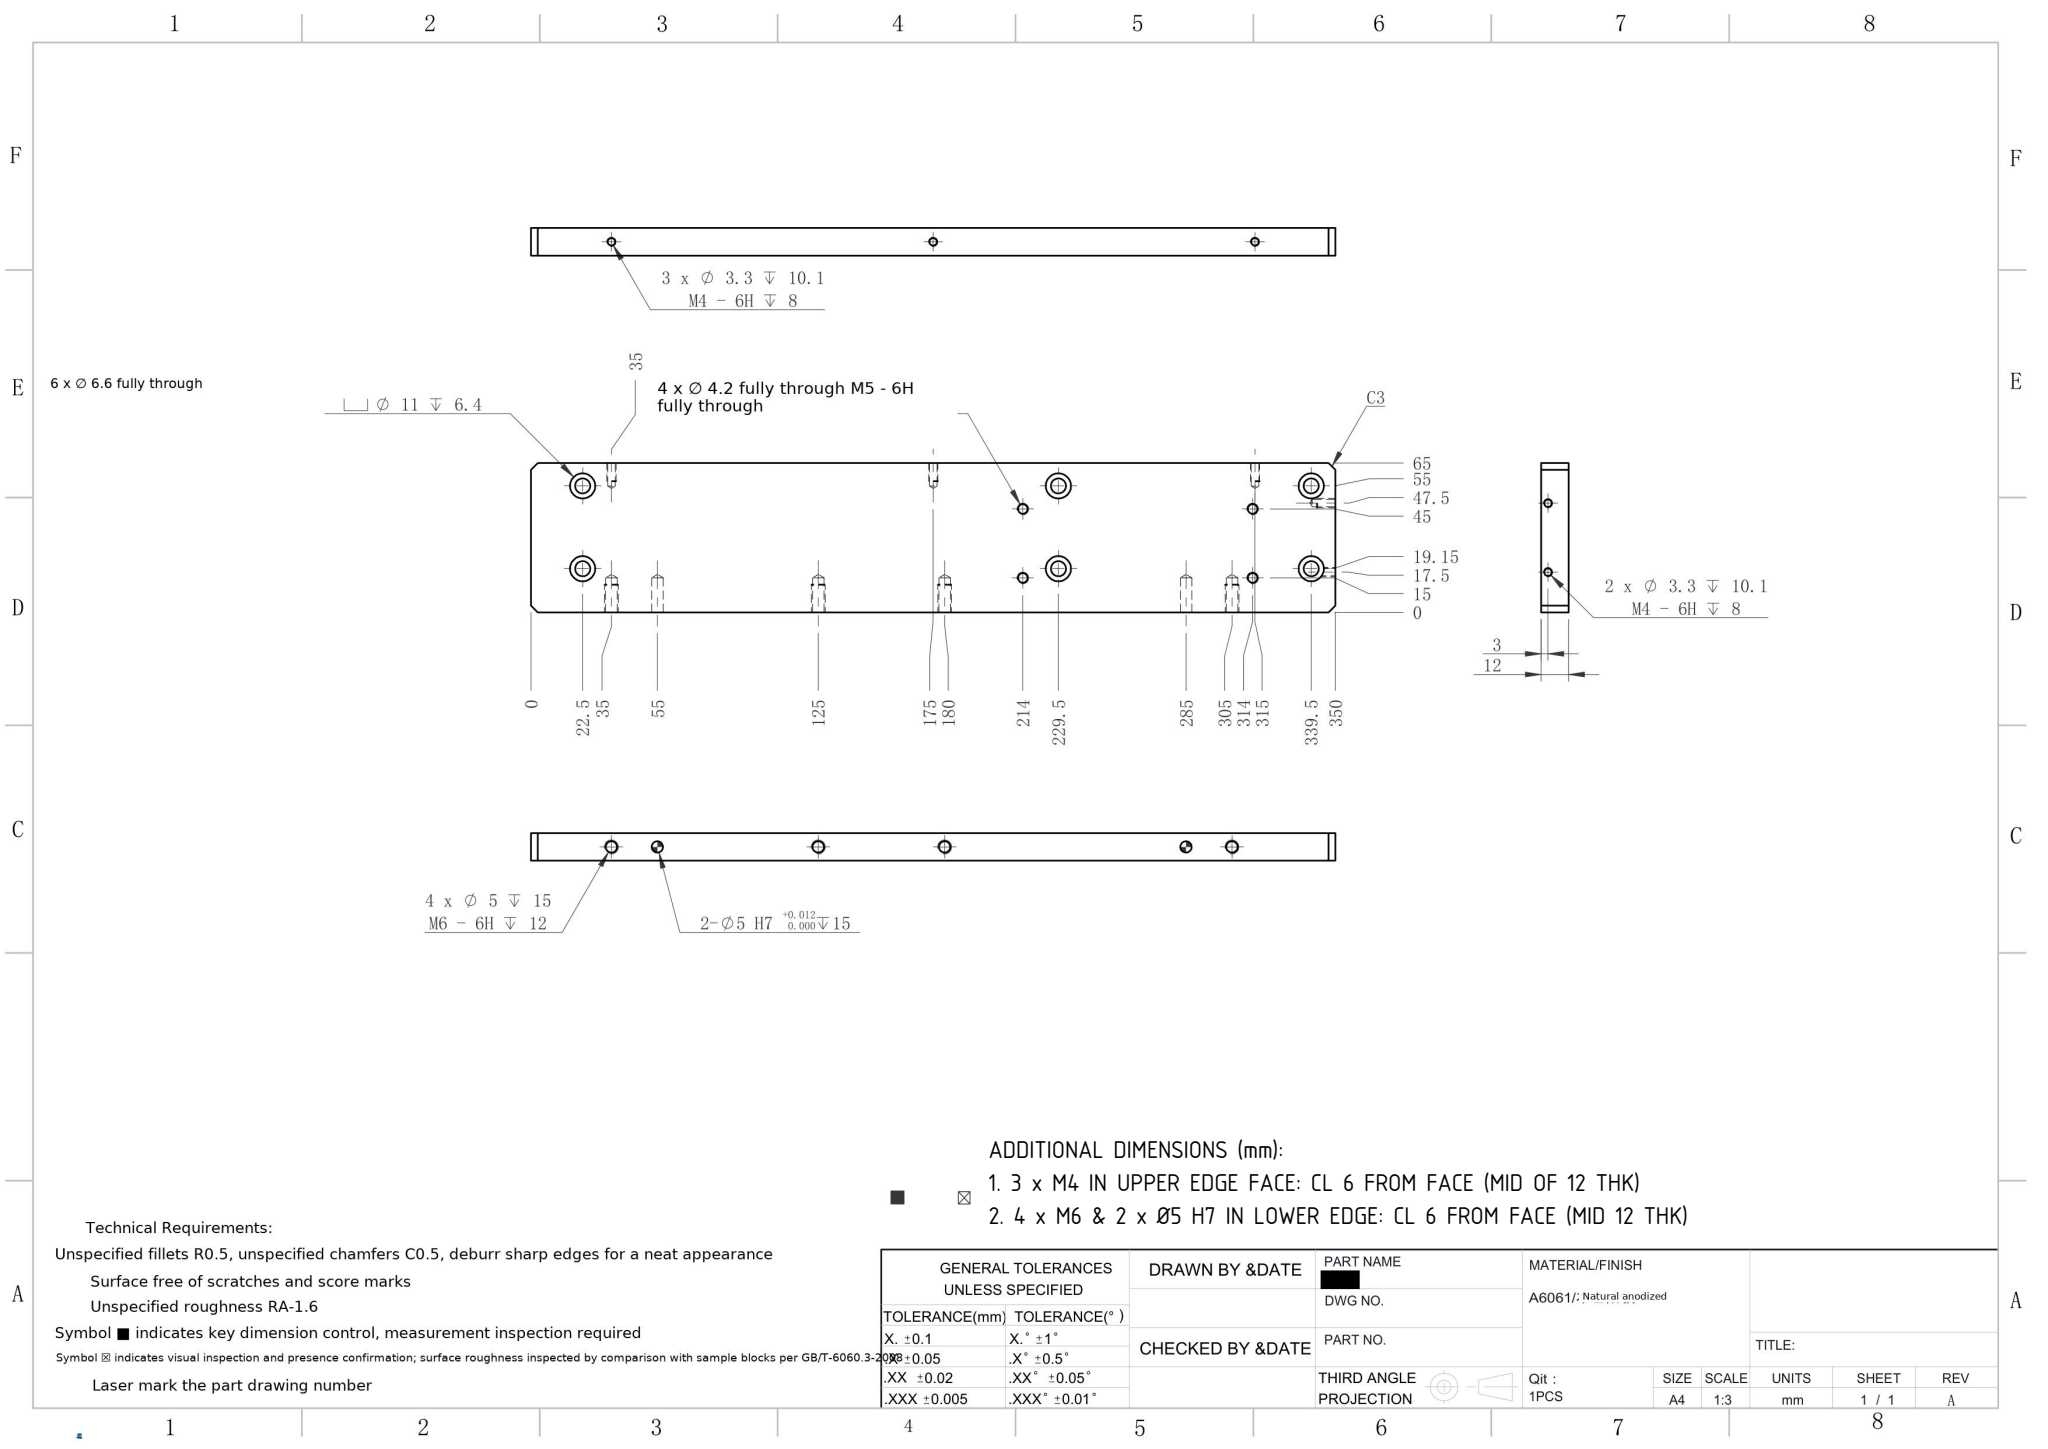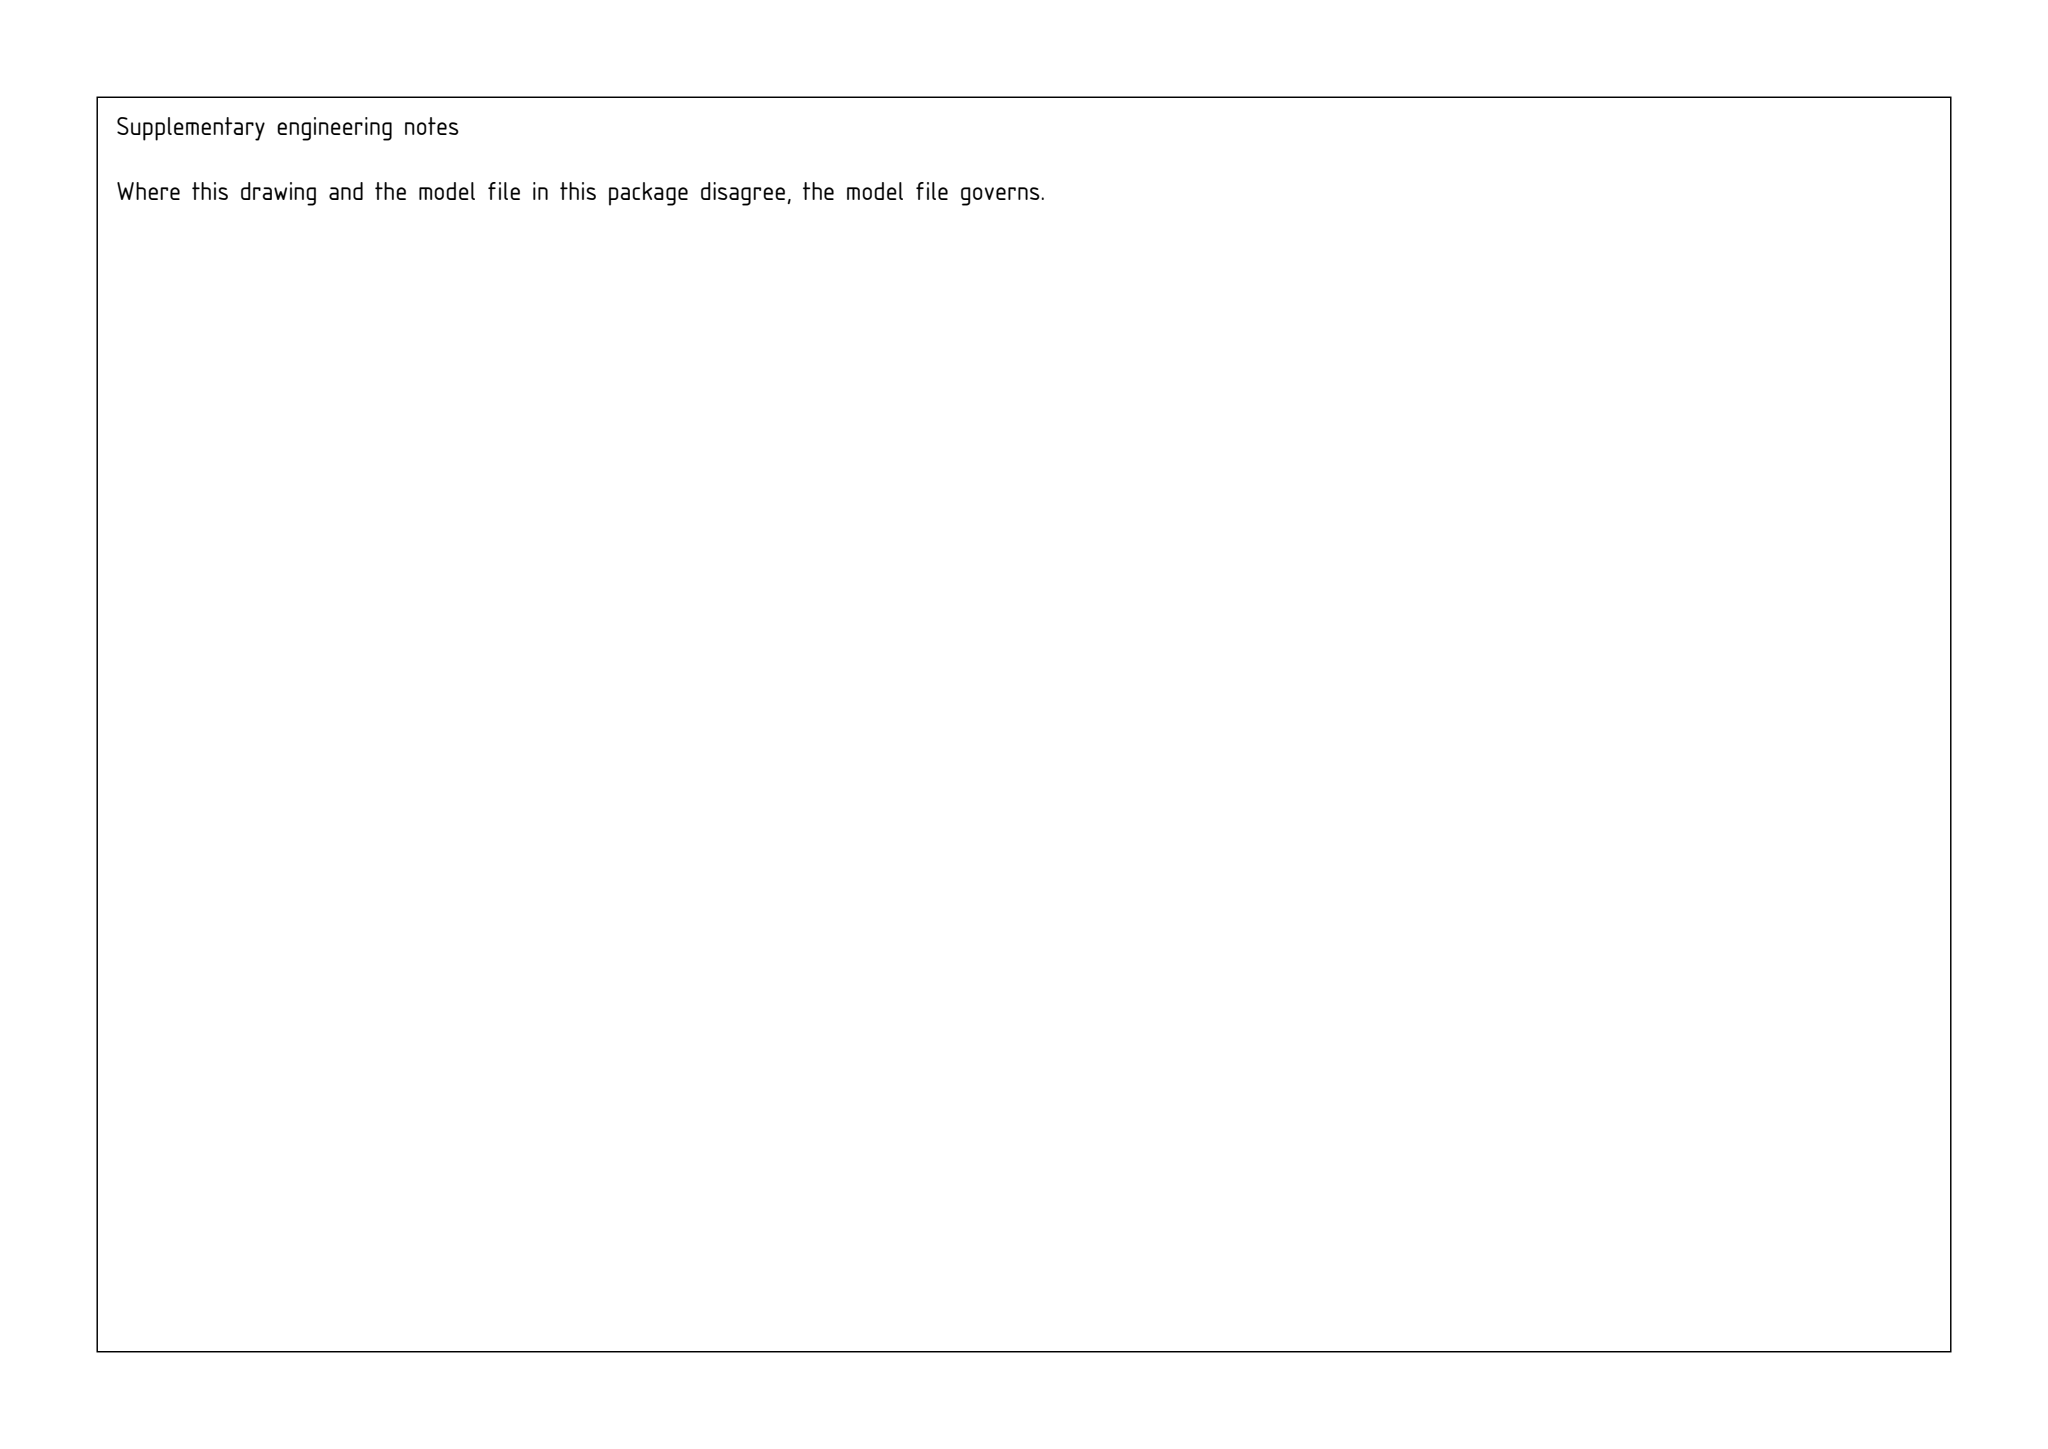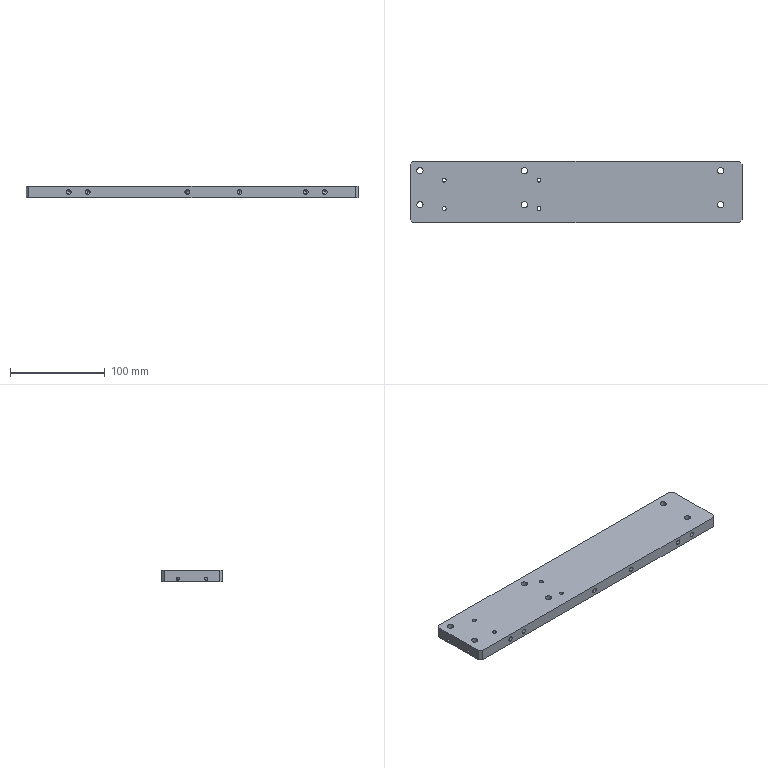Part | SolidWorks | mm | 1 solid | 90 faces | box 350 x 65 x 12 mm | volume 265092 mm3 | cylinder 54 | cone 20 | plane 16 | commonest cylinder face diameters 11 x12 6.6 x12 5 x12 3.3 x10 4.2 x8
build123d program:
from build123d import *

# Parameters (mm, degrees)
SKETCH1_W                                       = 350
SKETCH1_H                                       = 65
BOSS_EXTRUDE1_DEPTH                             = 12
CHAMFER1_SIZE                                   = 3
M4_TAPPED_HOLE1_D                               = 3.3
M4_TAPPED_HOLE1_DEPTH                           = 10.1
M4_TAPPED_HOLE1_TIP                             = 0.9914
M6_TAPPED_HOLE1_D                               = 5
M6_TAPPED_HOLE1_DEPTH                           = 15
M6_TAPPED_HOLE1_TIP                             = 1.502
SIZE_MM_DOWEL_PIN_HOLE_1_D                      = 5
SIZE_MM_DOWEL_PIN_HOLE_1_DEPTH                  = 15
SIZE_MM_DOWEL_PIN_HOLE_1_TIP                    = 1.502
M6_HEX_SOCKET_HEAD_CAP_SCREW_CBORE1_D           = 6.6
M6_HEX_SOCKET_HEAD_CAP_SCREW_CBORE1_CBORE_D     = 11
M6_HEX_SOCKET_HEAD_CAP_SCREW_CBORE1_CBORE_DEPTH = 6.4
M4_TAPPED_HOLE2_D                               = 3.3
M4_TAPPED_HOLE2_DEPTH                           = 10.1
M4_TAPPED_HOLE2_TIP                             = 0.9914
M5_TAPPED_HOLE1_D                               = 4.2


with BuildPart() as part:
    # Sketch1 → Boss-Extrude1 (new body)
    with BuildSketch(Plane.XY):
        Rectangle(SKETCH1_W, SKETCH1_H)
    extrude(amount=BOSS_EXTRUDE1_DEPTH)

    # Chamfer1
    chamfer1_edges = [part.edges().sort_by_distance(p)[0] for p in [
        (175, -32.5, 6),
        (-175, -32.5, 6),
        (-175, 32.5, 6),
        (175, 32.5, 6),
    ]]
    chamfer(chamfer1_edges, length=CHAMFER1_SIZE)

    # M4 Tapped Hole1
    with Locations(Plane(origin=(0, 32.5, 0), x_dir=(1, 0, 0), z_dir=(0, 1, 0))):
        with Locations((140, -6), (0, -6), (-140, -6)):
            Hole(M4_TAPPED_HOLE1_D / 2, depth=M4_TAPPED_HOLE1_DEPTH)
            with Locations((0, 0, -(M4_TAPPED_HOLE1_DEPTH + M4_TAPPED_HOLE1_TIP / 2))):  # 118° drill point
                Cone(0, M4_TAPPED_HOLE1_D / 2, M4_TAPPED_HOLE1_TIP, mode=Mode.SUBTRACT)

    # M6 Tapped Hole1
    with Locations(Plane(origin=(0, -32.5, 0), x_dir=(-1, 0, 0), z_dir=(0, -1, 0))):
        with Locations((130, -6), (5, -6), (-140, -6), (-50, -6)):
            Hole(M6_TAPPED_HOLE1_D / 2, depth=M6_TAPPED_HOLE1_DEPTH)
            with Locations((0, 0, -(M6_TAPPED_HOLE1_DEPTH + M6_TAPPED_HOLE1_TIP / 2))):  # 118° drill point
                Cone(0, M6_TAPPED_HOLE1_D / 2, M6_TAPPED_HOLE1_TIP, mode=Mode.SUBTRACT)

    # Size mm Dowel Pin Hole 1
    with Locations(Plane(origin=(0, -32.5, 0), x_dir=(-1, 0, 0), z_dir=(0, -1, 0))):
        with Locations((-120, -6), (110, -6)):
            Hole(SIZE_MM_DOWEL_PIN_HOLE_1_D / 2, depth=SIZE_MM_DOWEL_PIN_HOLE_1_DEPTH)
            with Locations((0, 0, -(SIZE_MM_DOWEL_PIN_HOLE_1_DEPTH + SIZE_MM_DOWEL_PIN_HOLE_1_TIP / 2))):  # 118° drill point
                Cone(0, SIZE_MM_DOWEL_PIN_HOLE_1_D / 2, SIZE_MM_DOWEL_PIN_HOLE_1_TIP, mode=Mode.SUBTRACT)

    # M6 Hex Socket Head Cap Screw CBORE1 (through all)
    with Locations(Plane(origin=(0, 0, 0), x_dir=(-1, 0, 0), z_dir=(0, 0, -1))):
        with Locations((-152.5, 22.5), (-152.5, -13.5), (54.5, 22.5), (54.5, -13.5), (164.5, -13.5), (164.5, 22.5)):
            CounterBoreHole(M6_HEX_SOCKET_HEAD_CAP_SCREW_CBORE1_D / 2, M6_HEX_SOCKET_HEAD_CAP_SCREW_CBORE1_CBORE_D / 2, M6_HEX_SOCKET_HEAD_CAP_SCREW_CBORE1_CBORE_DEPTH)

    # M4 Tapped Hole2
    with Locations(Plane.ZY.offset(175)):
        with Locations((3, 15), (3, -15)):
            Hole(M4_TAPPED_HOLE2_D / 2, depth=M4_TAPPED_HOLE2_DEPTH)
            with Locations((0, 0, -(M4_TAPPED_HOLE2_DEPTH + M4_TAPPED_HOLE2_TIP / 2))):  # 118° drill point
                Cone(0, M4_TAPPED_HOLE2_D / 2, M4_TAPPED_HOLE2_TIP, mode=Mode.SUBTRACT)

    # M5 Tapped Hole1 (through all)
    with Locations(Plane(origin=(0, 0, 0), x_dir=(-1, 0, 0), z_dir=(0, 0, -1))):
        with Locations((39, 12.5), (39, -17.5), (139, -17.5), (139, 12.5)):
            Hole(M5_TAPPED_HOLE1_D / 2)


solid = part.part